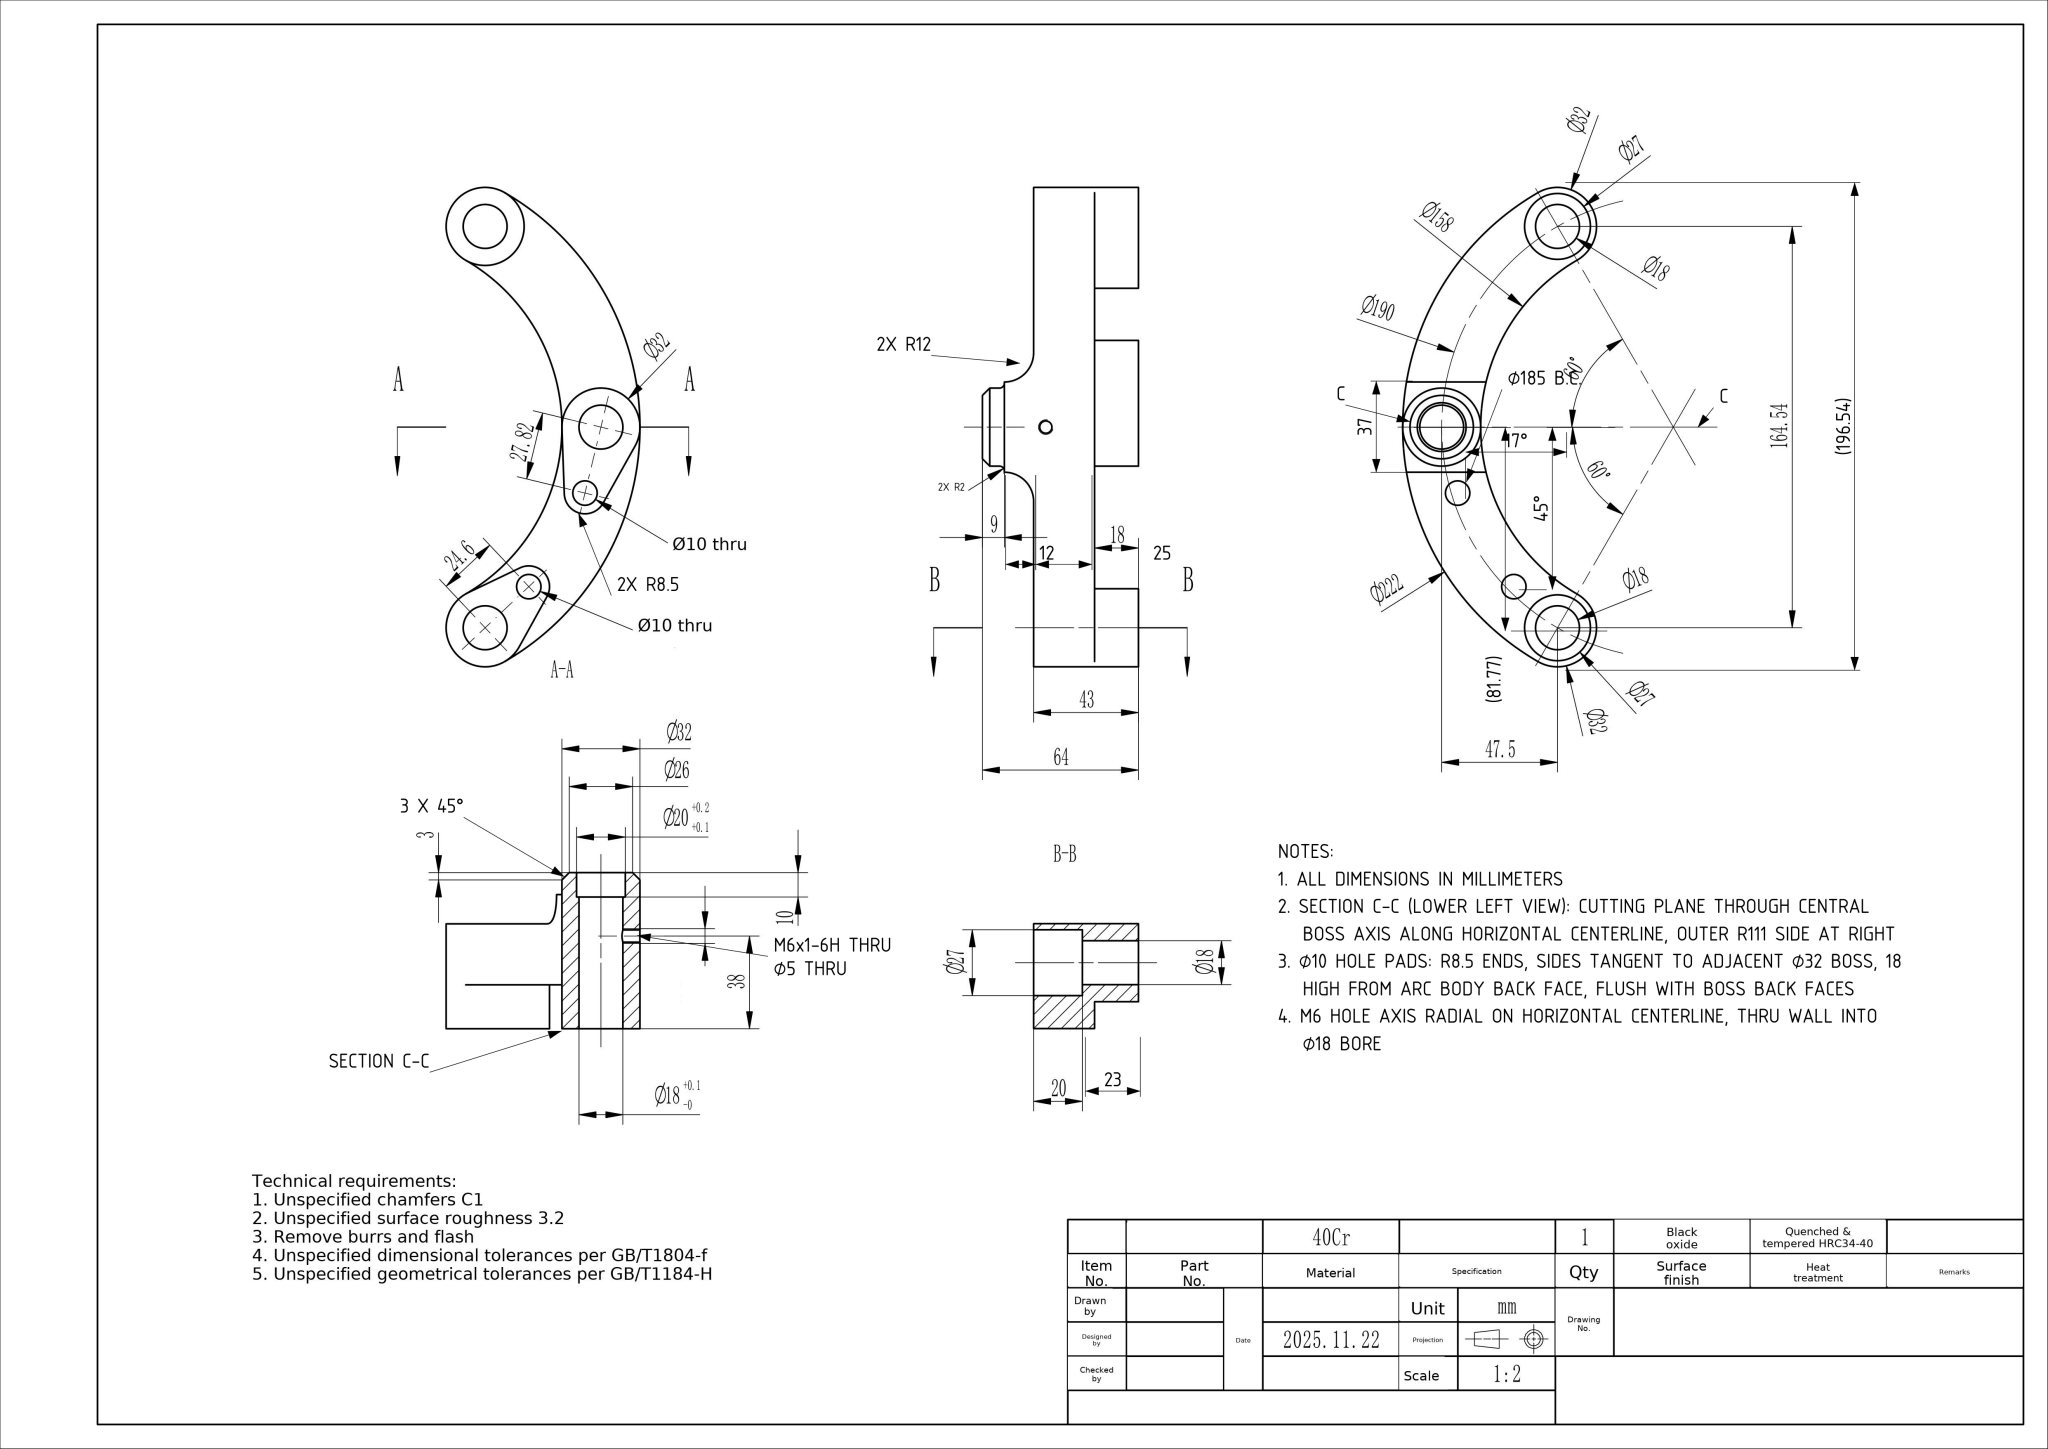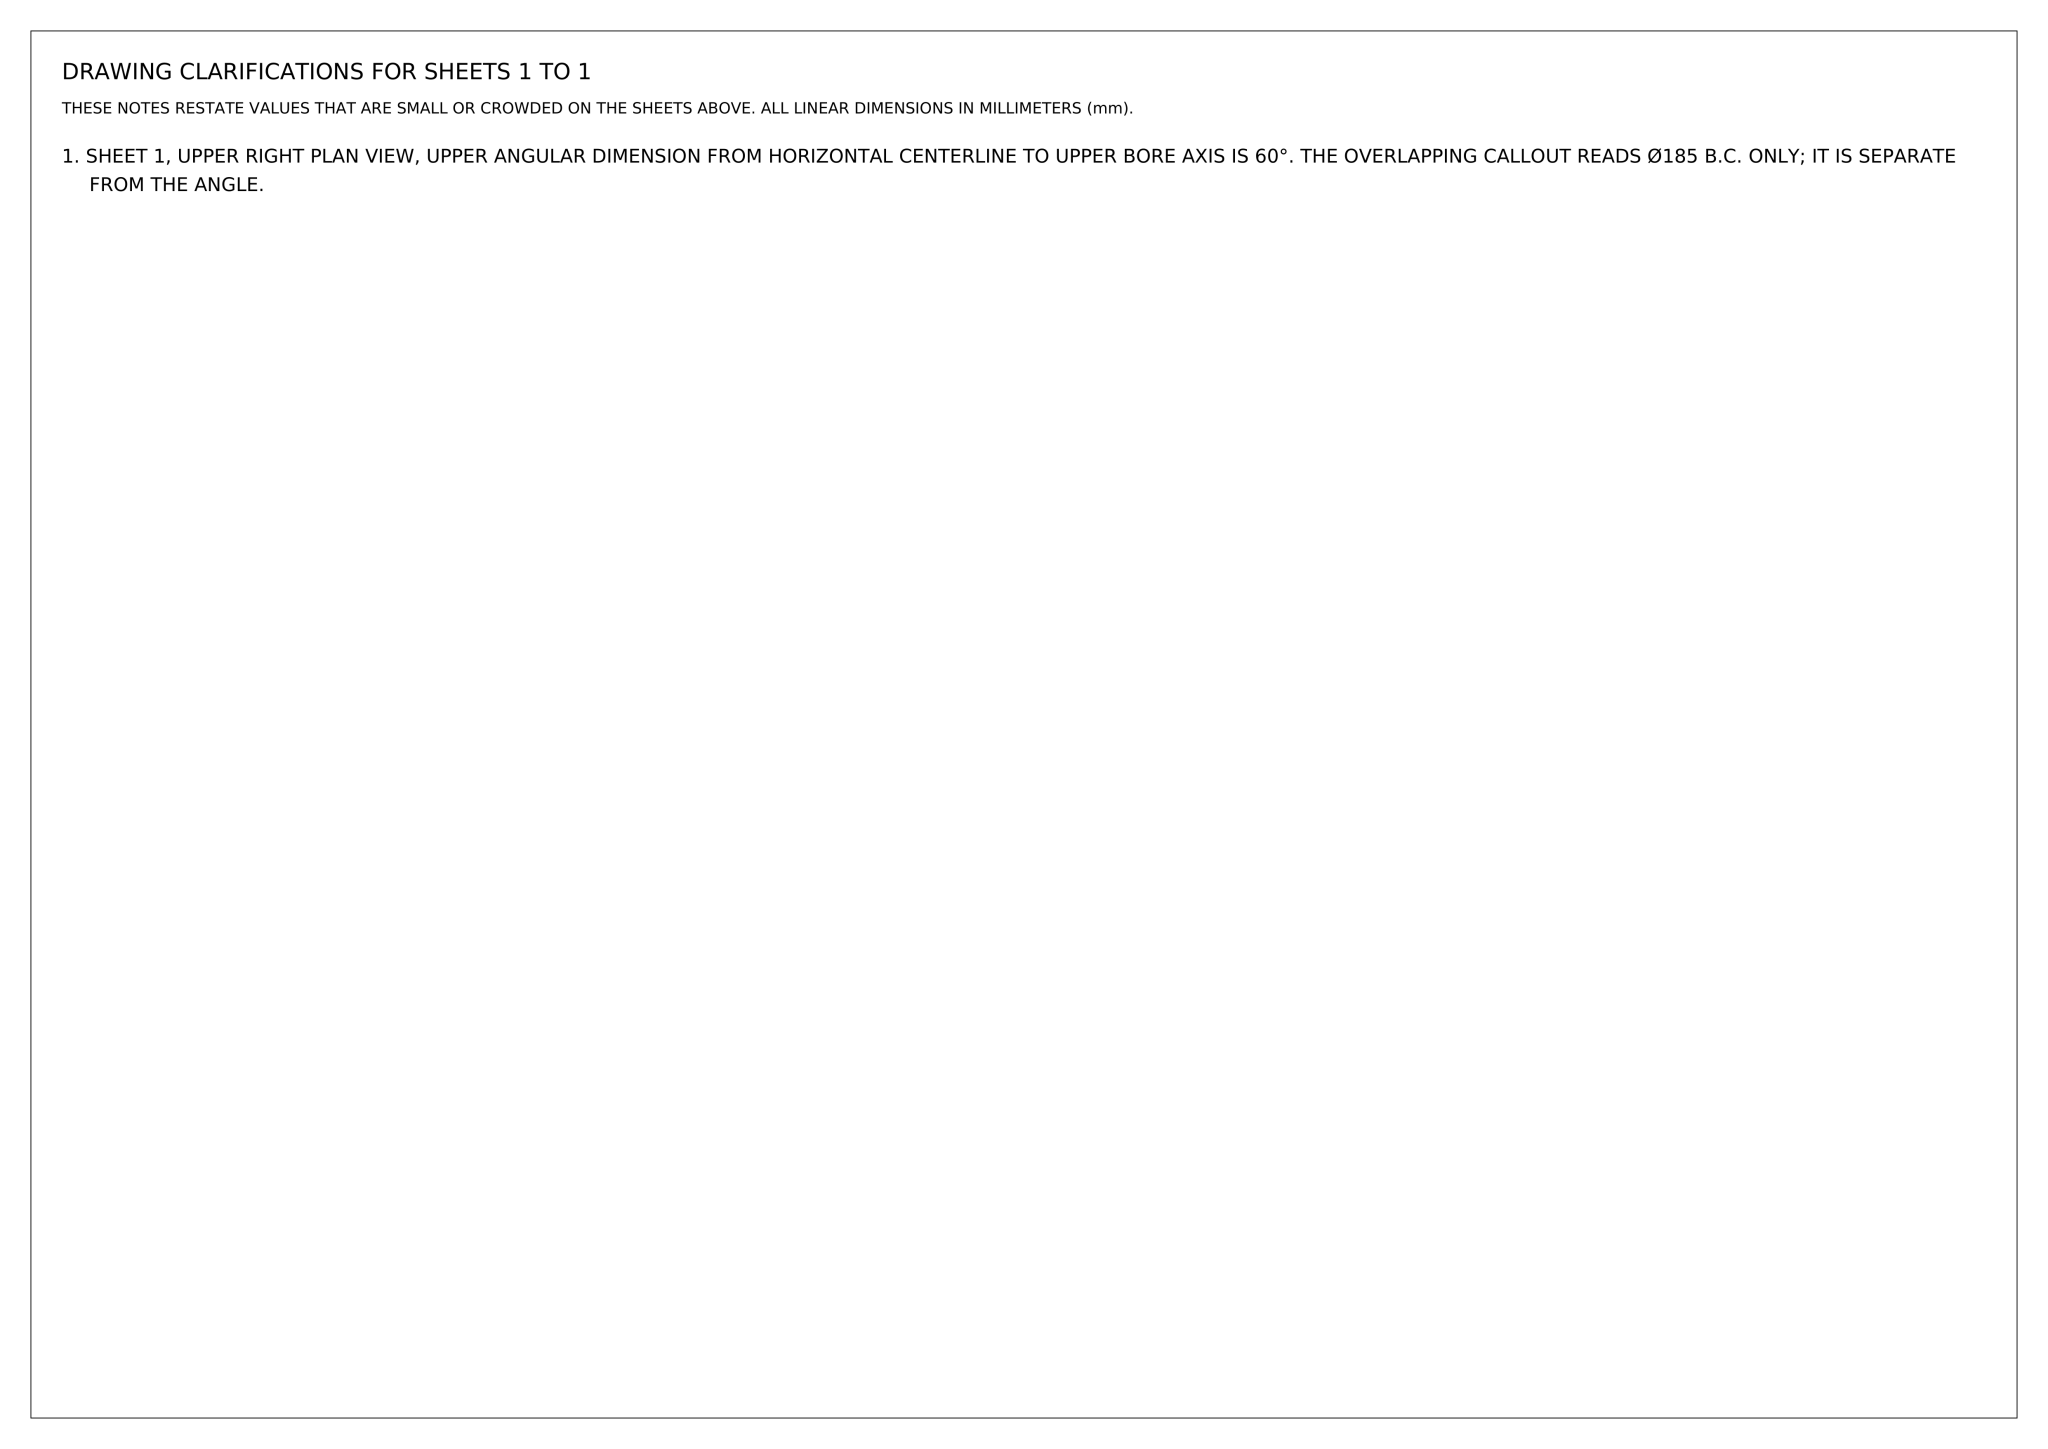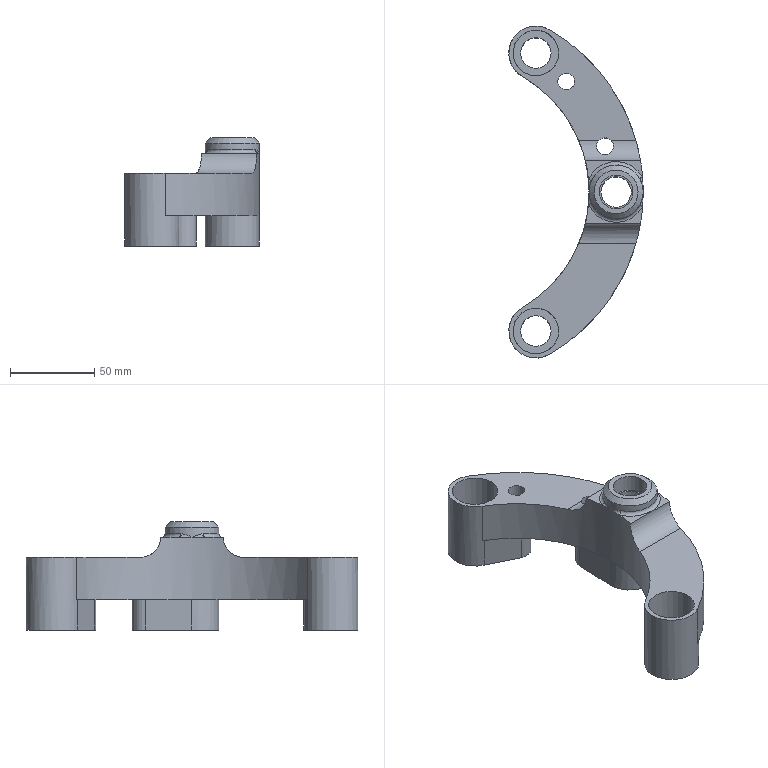Part | NX | mm | 1 solid | 43 faces | box 79.5 x 196.54 x 64 mm | volume 201168 mm3 | cylinder 19 | plane 17 | spline 4 | torus 2 | cone 1 | commonest cylinder face diameters 32 x4 18 x3 27 x2 10 x2 24 x2 17 x2 158 x1 222 x1